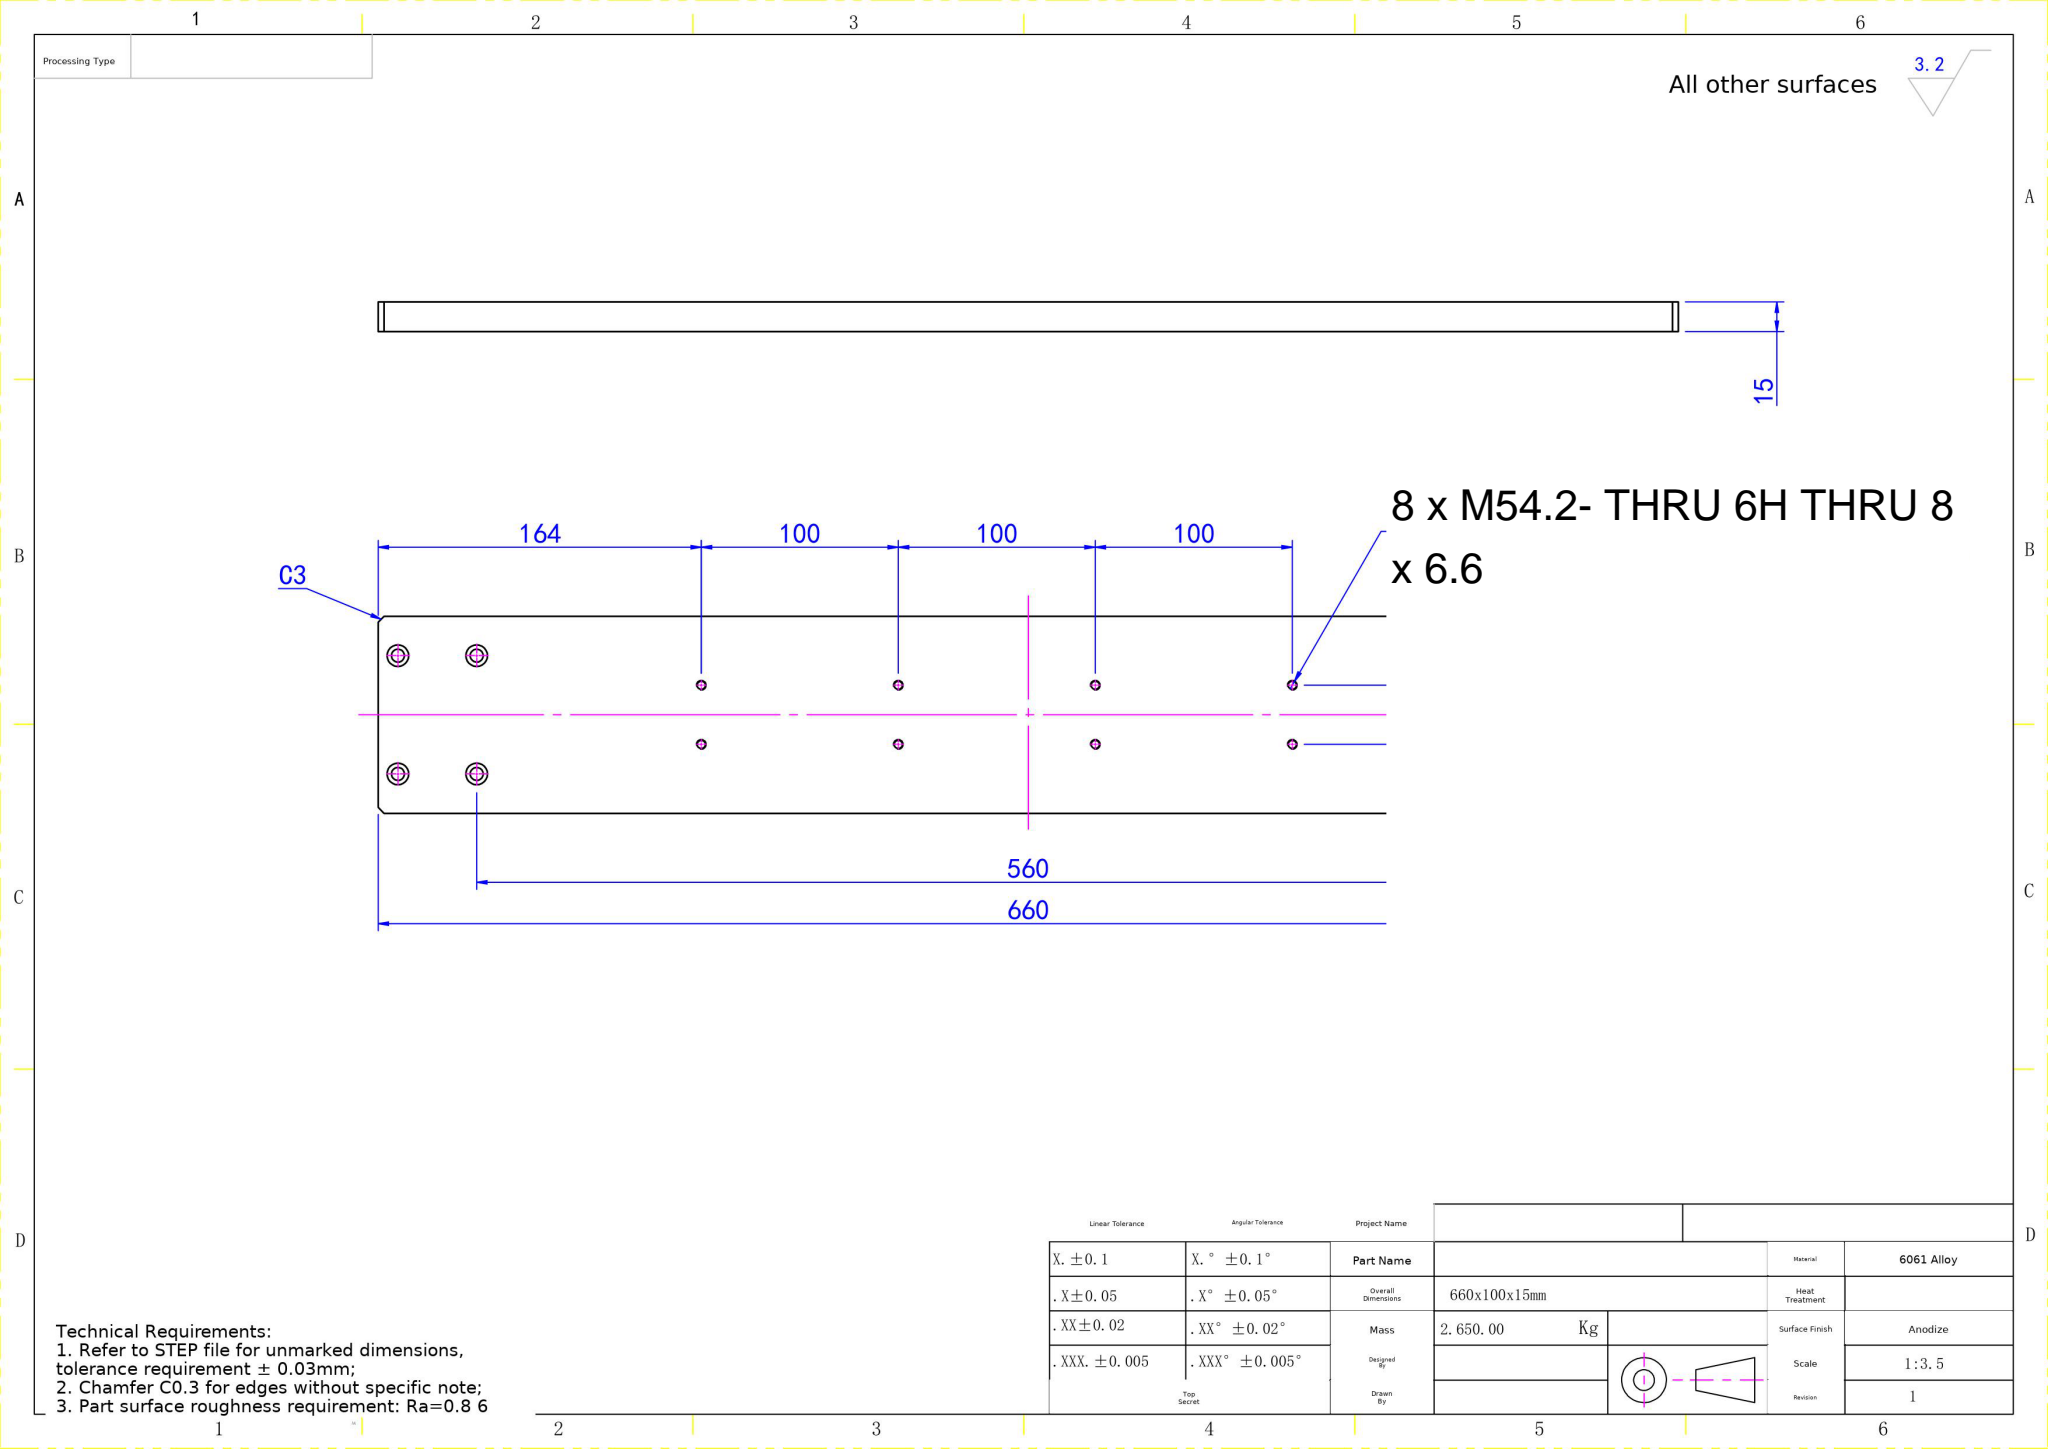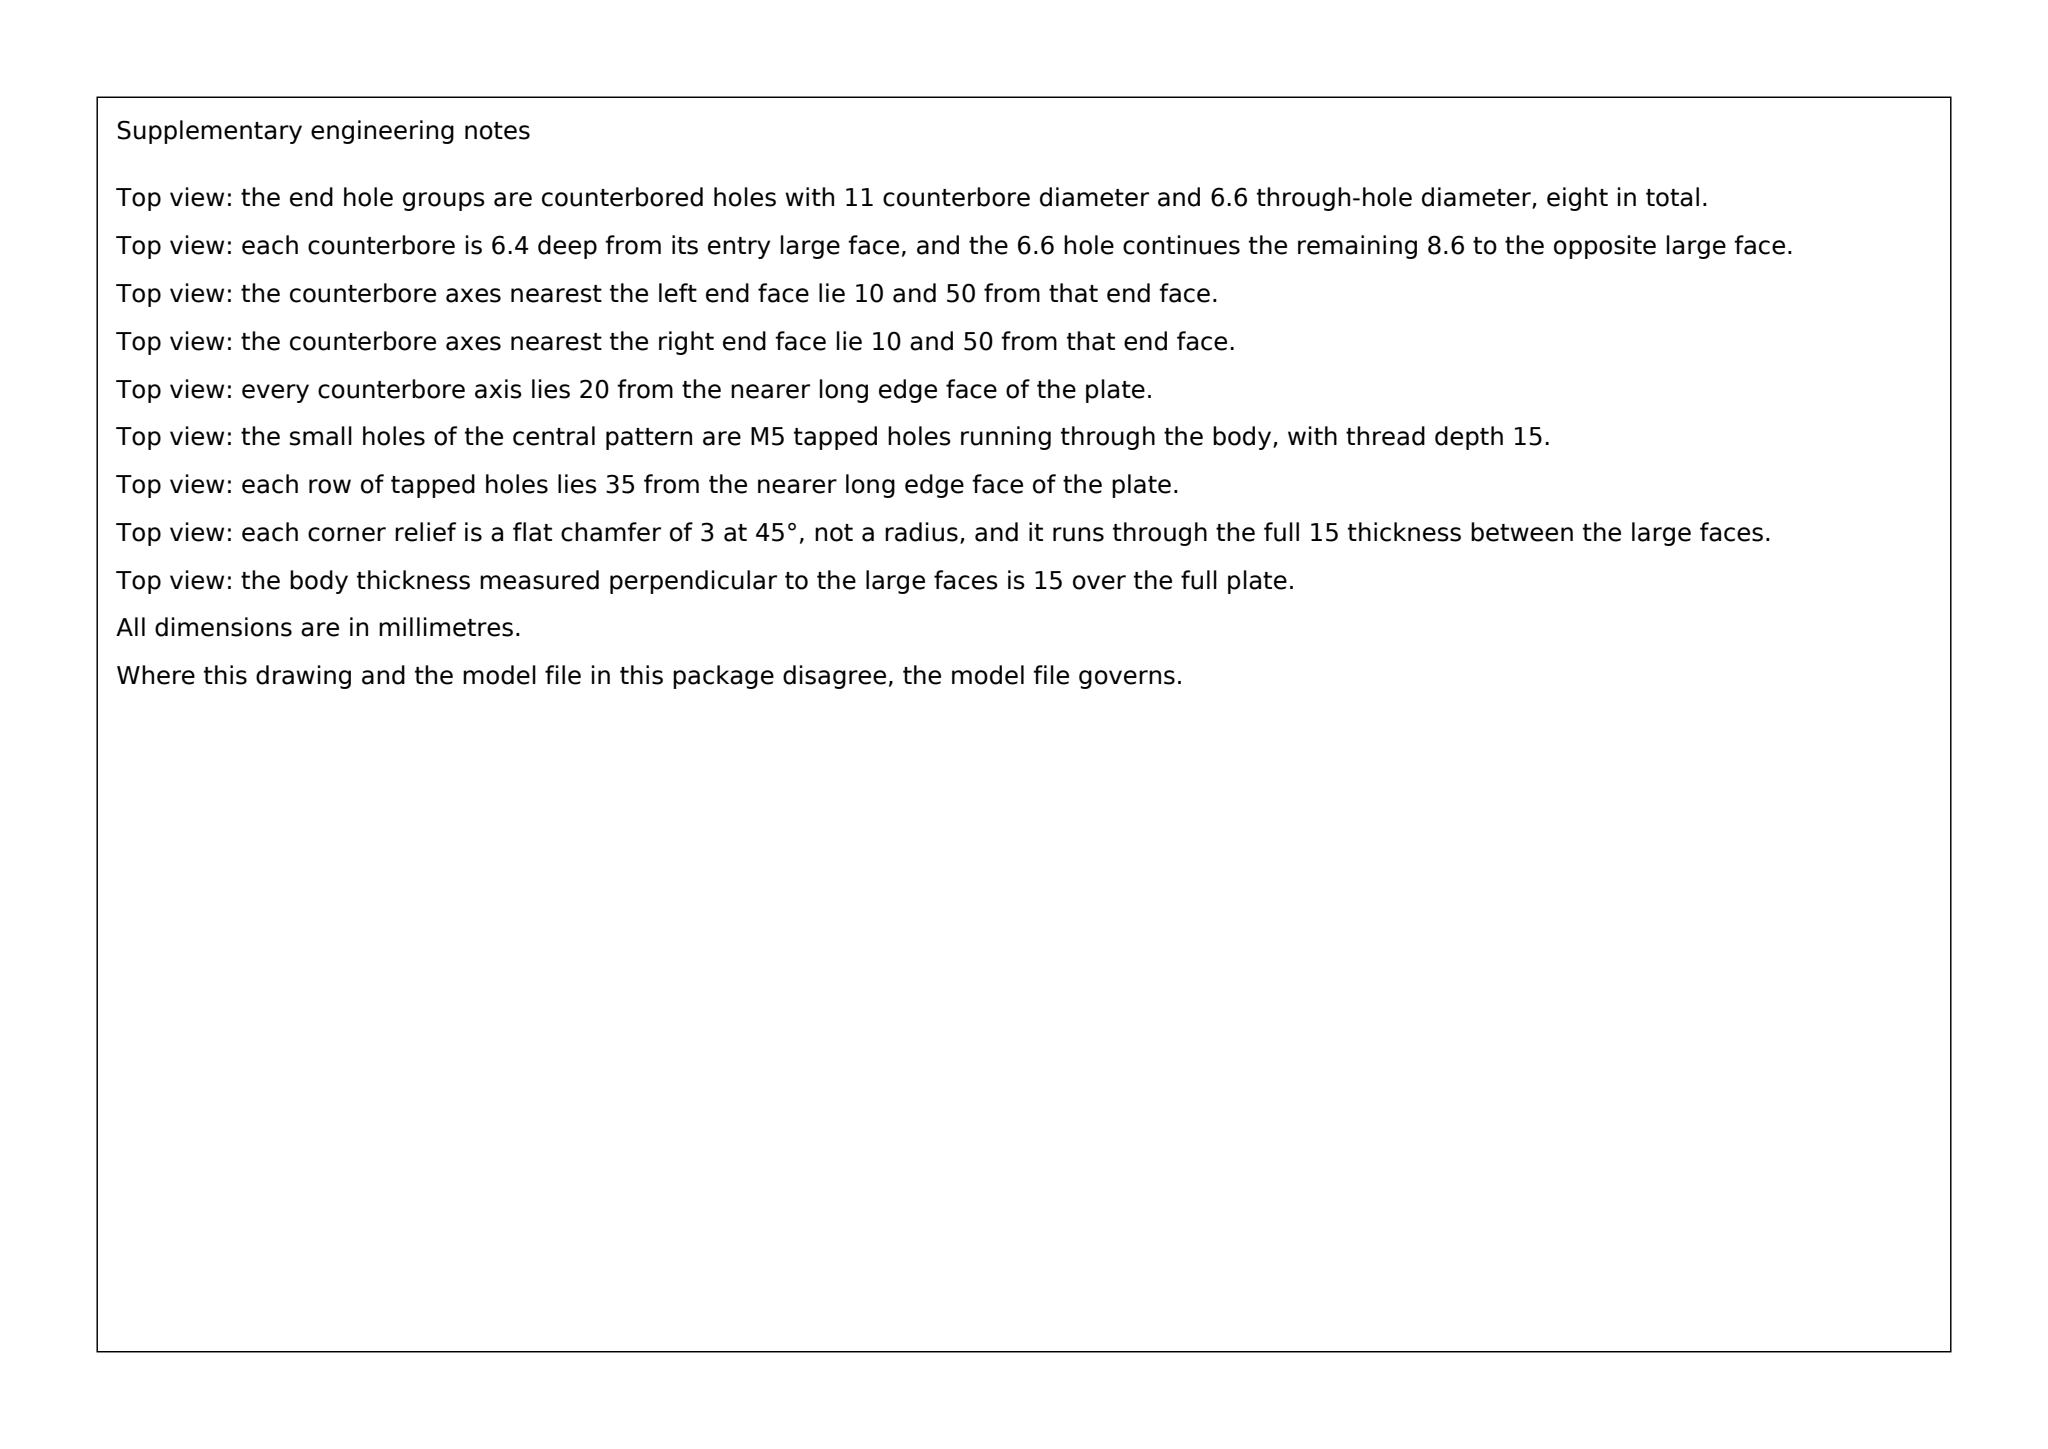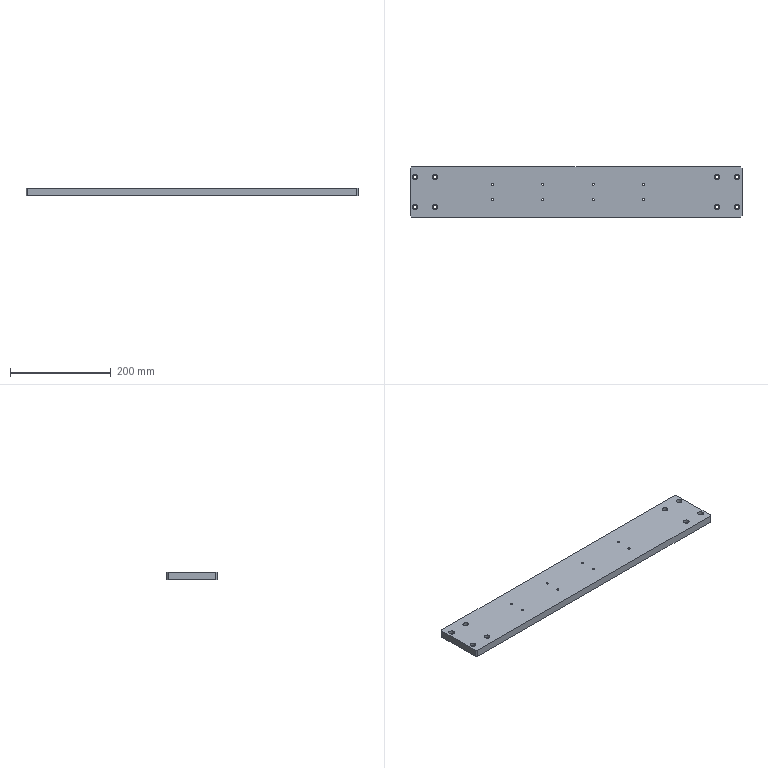Part | SolidWorks | mm | 1 solid | 66 faces | box 660 x 100 x 15 mm | volume 980848 mm3 | cylinder 48 | plane 18 | commonest cylinder face diameters 4.2 x16 11 x16 6.6 x16
Drawing notes:
8X Ø4.2 THRU (15 thk), hole centers at X=164, 264, 364, 464 from left end face; Y=35 and Y=65 from bottom long edge | from the solid: cylinders[4.2,z,(164/264/364/464, 35 and 65),length 15] x8
8X Ø6.6 THRU, C'BORE Ø11 DP 6.4 from top face; centers at X=10, 50, 610, 650 from left end face; Y=20 and Y=80 from bottom long edge | from the solid: cylinders[6.6,z,len 8.6] and [11.0,z,len 6.4] at (10/50/610/650, 20 and 80)
8X Ø4.2 THRU (15 mm thickness), 2 rows at Y=35 and Y=65 from bottom edge; X=164, 264, 364, 464 from left end | from the solid: cylinders dia 4.2, axis z, length 15.0 at (164/264/364/464, 35 and 65)
8X Ø6.6 THRU-type hole DP 8.6 with CBORE Ø11 DP 6.4 from top face; X=10, 50, 610, 650 and Y=20, 80 from the lower-left corner | from the solid: cylinders dia 6.6 len 8.6 and dia 11.0 len 6.4 at (10/50/610/650, 20/80); plane z=8.6
build123d program:
from build123d import *

# Parameters (mm, degrees)
SKETCH1_W                                       = 660
SKETCH1_H                                       = 100
BOSS_EXTRUDE1_DEPTH                             = 15
M6_HEX_SOCKET_HEAD_CAP_SCREW_CBORE4_D           = 6.6
M6_HEX_SOCKET_HEAD_CAP_SCREW_CBORE4_CBORE_D     = 11
M6_HEX_SOCKET_HEAD_CAP_SCREW_CBORE4_CBORE_DEPTH = 6.4
CHAMFER1_SIZE                                   = 3
M5_TAPPED_HOLE1_D                               = 4.2


with BuildPart() as part:
    # Sketch1 → Boss-Extrude1 (new body)
    with BuildSketch(Plane.XY):
        with Locations((330, 50)):
            Rectangle(SKETCH1_W, SKETCH1_H)
    extrude(amount=BOSS_EXTRUDE1_DEPTH)

    # M6 Hex Socket Head Cap Screw CBORE4 (through all)
    with Locations(Plane.XY.offset(15)):
        with Locations((610, 80), (650, 80), (650, 20), (610, 20), (50, 20), (10, 20), (10, 80), (50, 80)):
            CounterBoreHole(M6_HEX_SOCKET_HEAD_CAP_SCREW_CBORE4_D / 2, M6_HEX_SOCKET_HEAD_CAP_SCREW_CBORE4_CBORE_D / 2, M6_HEX_SOCKET_HEAD_CAP_SCREW_CBORE4_CBORE_DEPTH)

    # Chamfer1
    chamfer1_edges = [part.edges().sort_by_distance(p)[0] for p in [
        (0, 100, 7.5),
        (660, 100, 7.5),
        (660, 0, 7.5),
        (0, 0, 7.5),
    ]]
    chamfer(chamfer1_edges, length=CHAMFER1_SIZE)

    # M5 Tapped Hole1 (through all)
    with Locations(Plane(origin=(0, 0, 0), x_dir=(-1, 0, 0), z_dir=(0, 0, -1))):
        with Locations((-264, 65), (-264, 35), (-364, 65), (-364, 35), (-164, 65), (-164, 35), (-464, 65), (-464, 35)):
            Hole(M5_TAPPED_HOLE1_D / 2)


solid = part.part